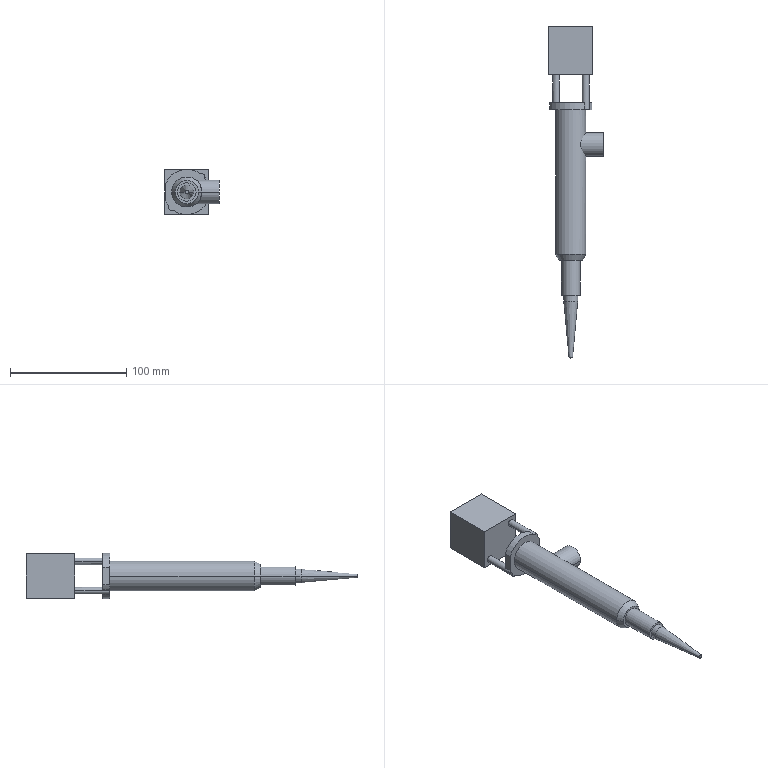Component | SolidWorks | RubberHead-2 | 4 solids | 41 faces | volume 151559 mm3 | plane 19 | cylinder 18 | cone 4 | commonest cylinder face diameters 20 x4 6 x4 39 x4 26 x2 12 x2 16 x2